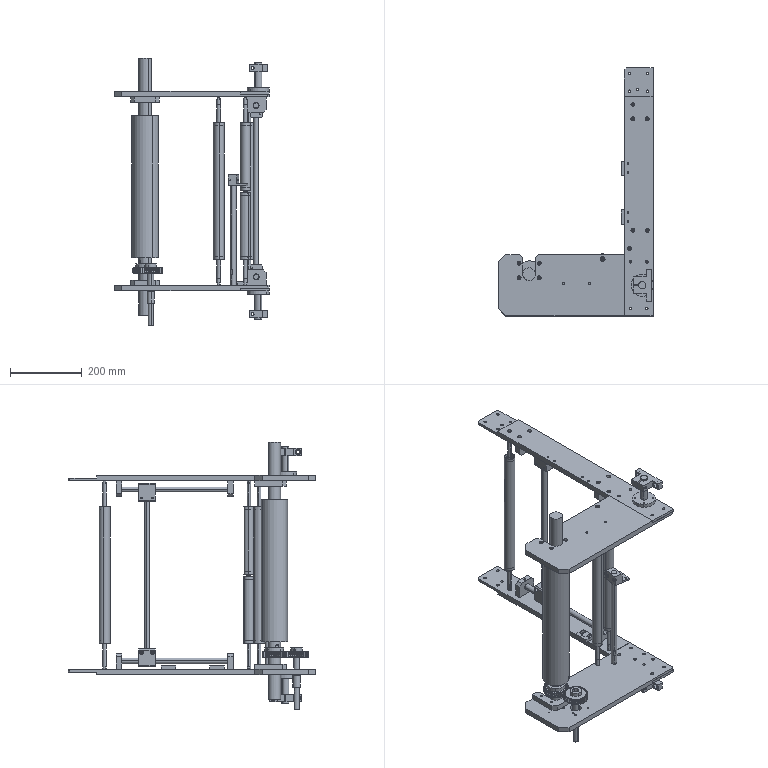Assembly | SolidWorks | mm | 34 component files | 34 solids | 1507 faces | box 431 x 690 x 744.77 mm | volume 6762911 mm3 | cylinder 825 | plane 364 | cone 318 | commonest cylinder face diameters 7 x110 5 x107 24.415 x68 24.155 x68 68 x66 59 x64 11 x50 8.5 x36
Bill of materials:
AirShaft | 1 |  | Stepped cylindrical shaft: a long central large-diameter section with smaller-diameter journals extending from both ends; one end journal has a narrow circumferential groove near the shoulder.
BottomPlate(1) | 1 |  | Flat rectangular plate with two chamfered corners at one end, an open U-shaped slot entering from that end, several through holes, and a stepped thinner region at the opposite end carrying a grid of holes.
BottomPlate(2) | 1 |  | Flat rectangular plate similar in outline to a slotted plate: chamfered corners, open U-slot at one end, a large round through hole with a ring of small holes near the slot, scattered small holes, and a grid of holes at the opposite end; thickness step appears on the underside at that end.
ConnectionAxis | 1 |  | Stepped cylindrical pin with a short larger-diameter collar between two smaller shank sections of slightly different diameters; one end has a small central axial hole, ends are chamfered.
ConnectionBase | 2 |  | Flanged post: a circular disc flange with four through holes on a bolt circle, joined to a solid cylindrical shank of smaller diameter.
Crossbar | 1 |  | Long slender plain cylindrical rod of constant diameter with flat ends.
FixedMount | 2 |  | T-shaped block: a long base bar with two horizontal through holes, and a perpendicular boss containing a large vertical through bore with a narrow slit running from the bore to the outer edge, plus a cross hole through the split portion.
Gear1 | 1 |  | Spur gear with straight teeth (roughly 30) and chamfered tips, an integral raised hub on one face, a large central bore with a keyway, and a small radial hole through the hub at the keyway.
Gear2 | 1 |  | Spur gear with straight teeth (roughly 30) and chamfered tips, a smaller-diameter raised hub, a relatively small central bore with keyway, and a small radial hole in the hub.
GuideRodMount | 4 |  | Rectangular block with two chamfered upper corners, a large round through bore through the main face, and a small chamfered hole in the top face (with a corresponding hole visible on the opposite face).
NameDuplicate-1Slider | 2 |  | Plain cylindrical rod/pin of constant diameter with small chamfers at both ends.
PhotoelectricMount | 2 |  | Rectangular block with two counterbored obround (slotted) through holes near one edge and two small chamfered round through holes near the opposite edge.
Roller1 | 2 |  | Long, straight, thin-walled cylindrical tube with a constant cross-section and a through bore.
RollerAxis1 | 2 |  | Very slender cylindrical rod or pin with a small axial hole at one end. The end view shows a conical recess, which suggests a blind or drilled hole with a pointed bottom.
Roller2 | 2 |  | Straight cylindrical tube with a through bore. It is shorter and thicker relative to its length than the other tubes in this set.
RollerAxis2 | 1 |  | Very slender cylindrical rod with a small axial hole at one end, a conical recess seen in the end view, and slightly reduced-diameter sections at both ends.
SlidingBearingHousing | 2 |  | Rectangular block with four chamfered long edges. It has one large cylindrical through bore along one axis and two smaller parallel through holes running perpendicular to it near the opposite end.
StopBlock | 2 |  | Flat U-shaped (fork) plate with a central slot that has a semicircular closed end. It has chamfered outer corners and four small through holes, two on each arm.
SupportRod | 1 |  | Solid slender cylindrical rod with flat ends and a small local feature near one end, possibly a cross hole, notch or flat.
SwitchMount | 1 |  | L-shaped block or bracket: a tall rectangular upright on one side of a thinner base flange. The upright has a large vertical through bore and two horizontal through holes; the flange has two small vertical through holes.
VerticalPlate(1) | 1 |  | Long, narrow flat plate with many through holes. Near one end there is a larger hole with four smaller holes around it; there are pairs of holes along the length and tiny holes near one long edge. The plate has a stepped or offset thickness profile, thicker in the middle, with the step on the side not visible in the isometric view.
VerticalPlate(2) | 1 |  | Long, narrow flat plate with the same hole pattern as unnamed part: a larger hole with four surrounding small holes near one end, pairs of holes along the length, and tiny holes near one edge. The stepped thickness profile is reversed, with a visible step on the top face.
Mates:
1. concentric | SlidingBearingHousing-1 face at (-36, 125.451, 205.5) dir (0, 0, -1) r 8 | Crossbar-1 face at (-36, 125.451, 219.68) dir (0, 0, -1) r 7
2. concentric | SlidingBearingHousing-1 face at (-36, 148.451, 238.5) dir (0, -1, 0) r 13 | NameDuplicate-1Slider-1 face at (-36, -103, 238.5) dir (0, 1, 0) r 8
3. concentric | SlidingBearingHousing-2 face at (-36, 125.451, -205.5) dir (0, 0, 1) r 8 | Crossbar-1 face at (-36, 125.451, 219.68) dir (0, 0, -1) r 7
4. concentric | SlidingBearingHousing-2 face at (-36, 148.451, -238.5) dir (0, -1, 0) r 13 | NameDuplicate-1Slider-2 face at (-36, 211, -238.5) dir (0, -1, 0) r 8